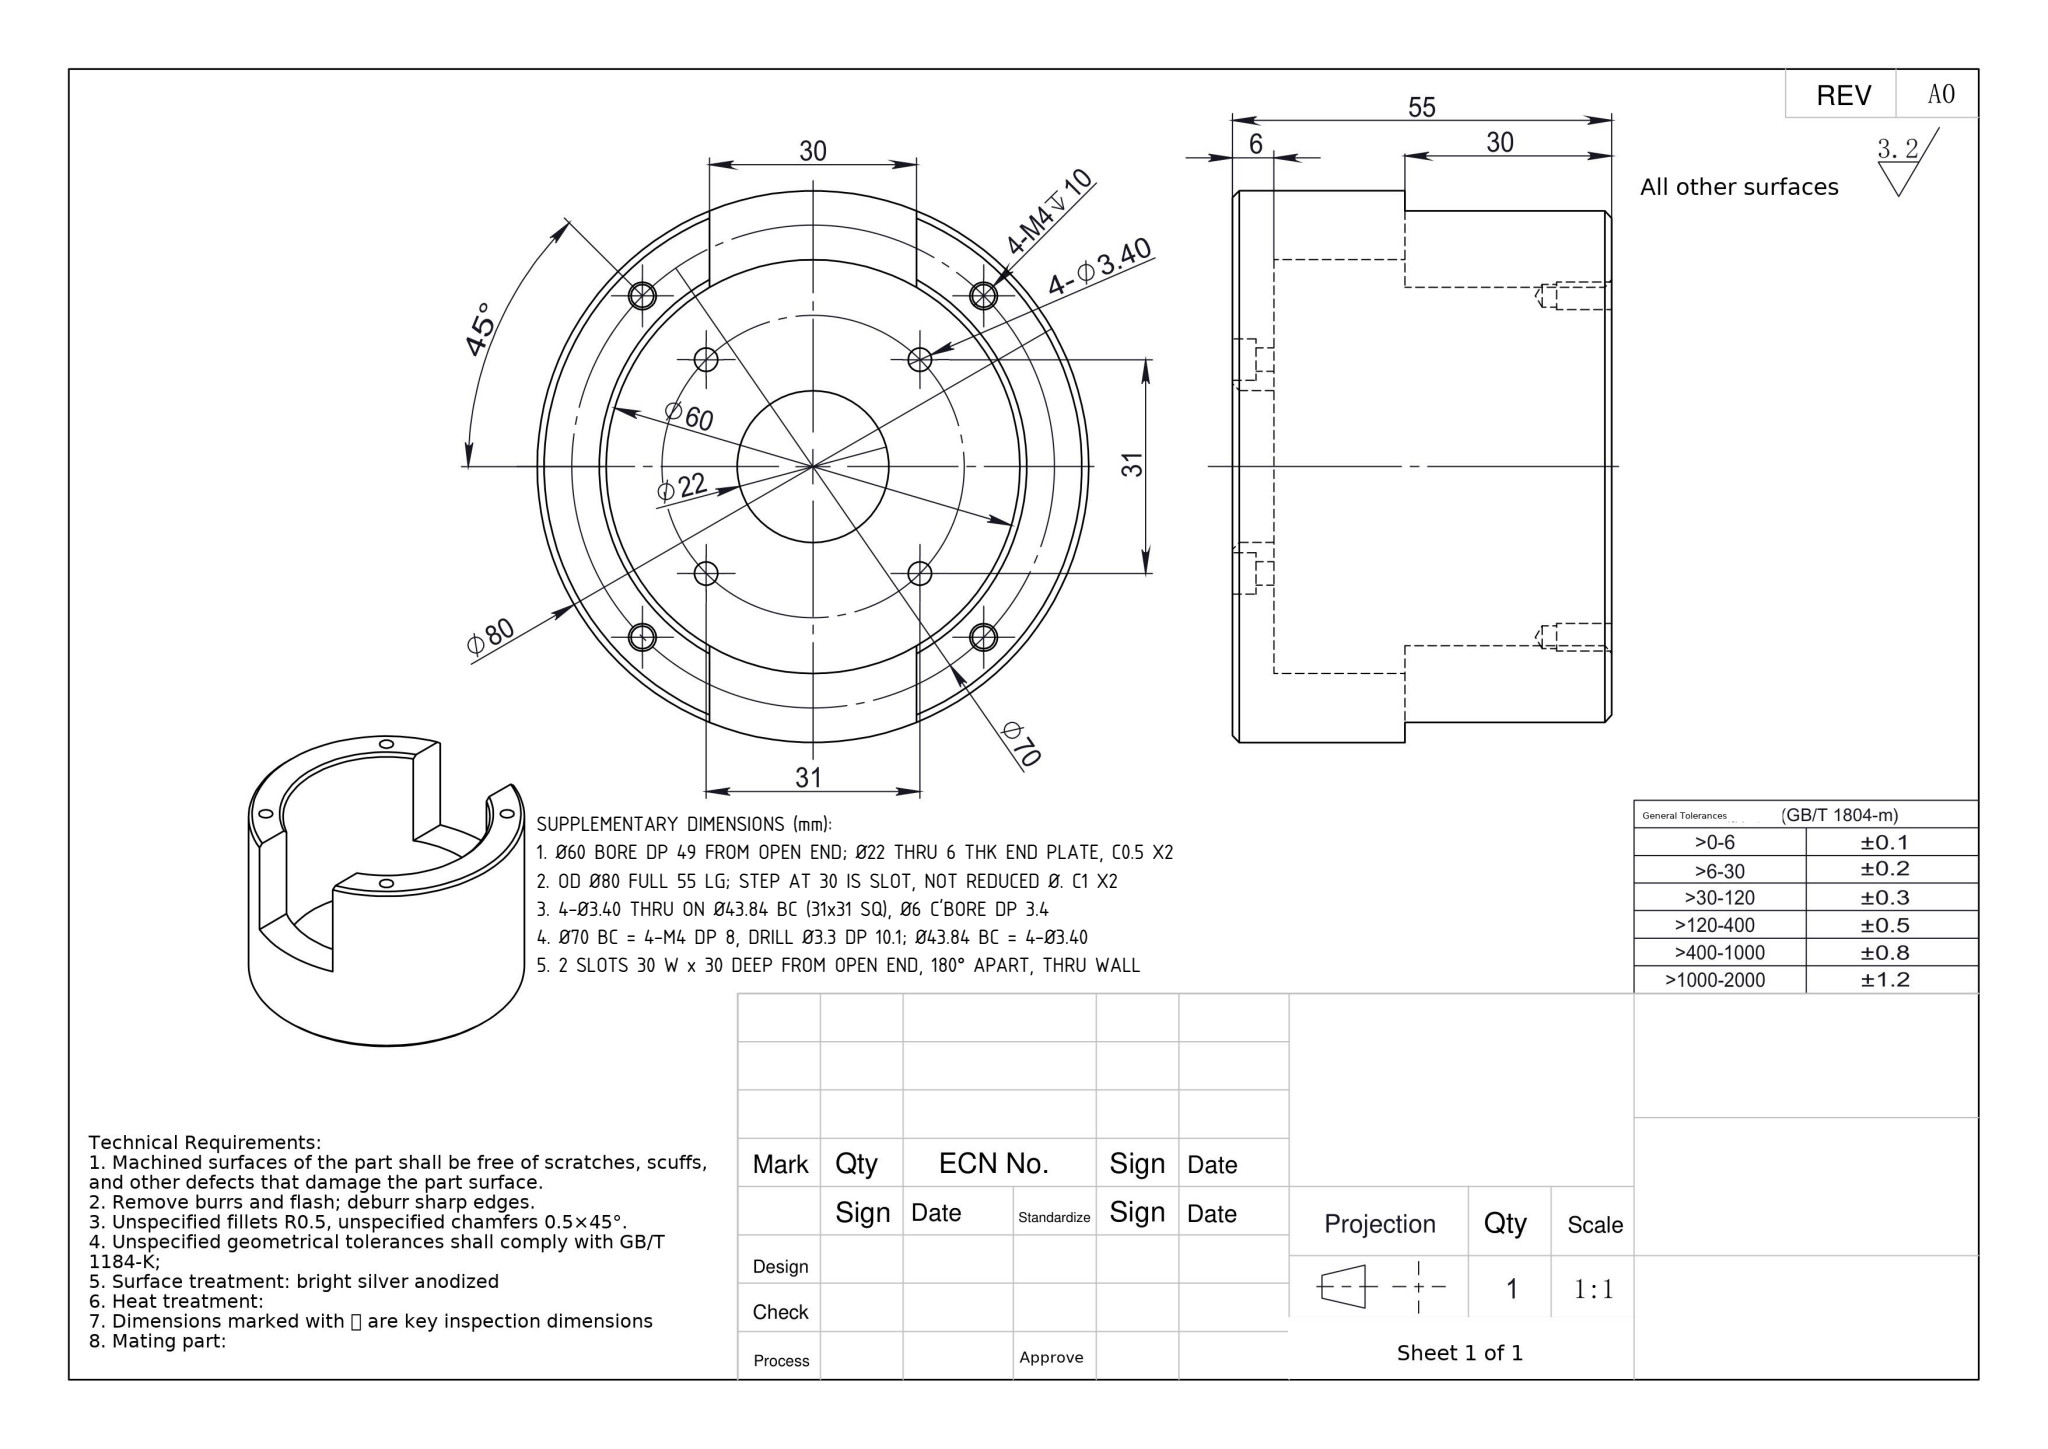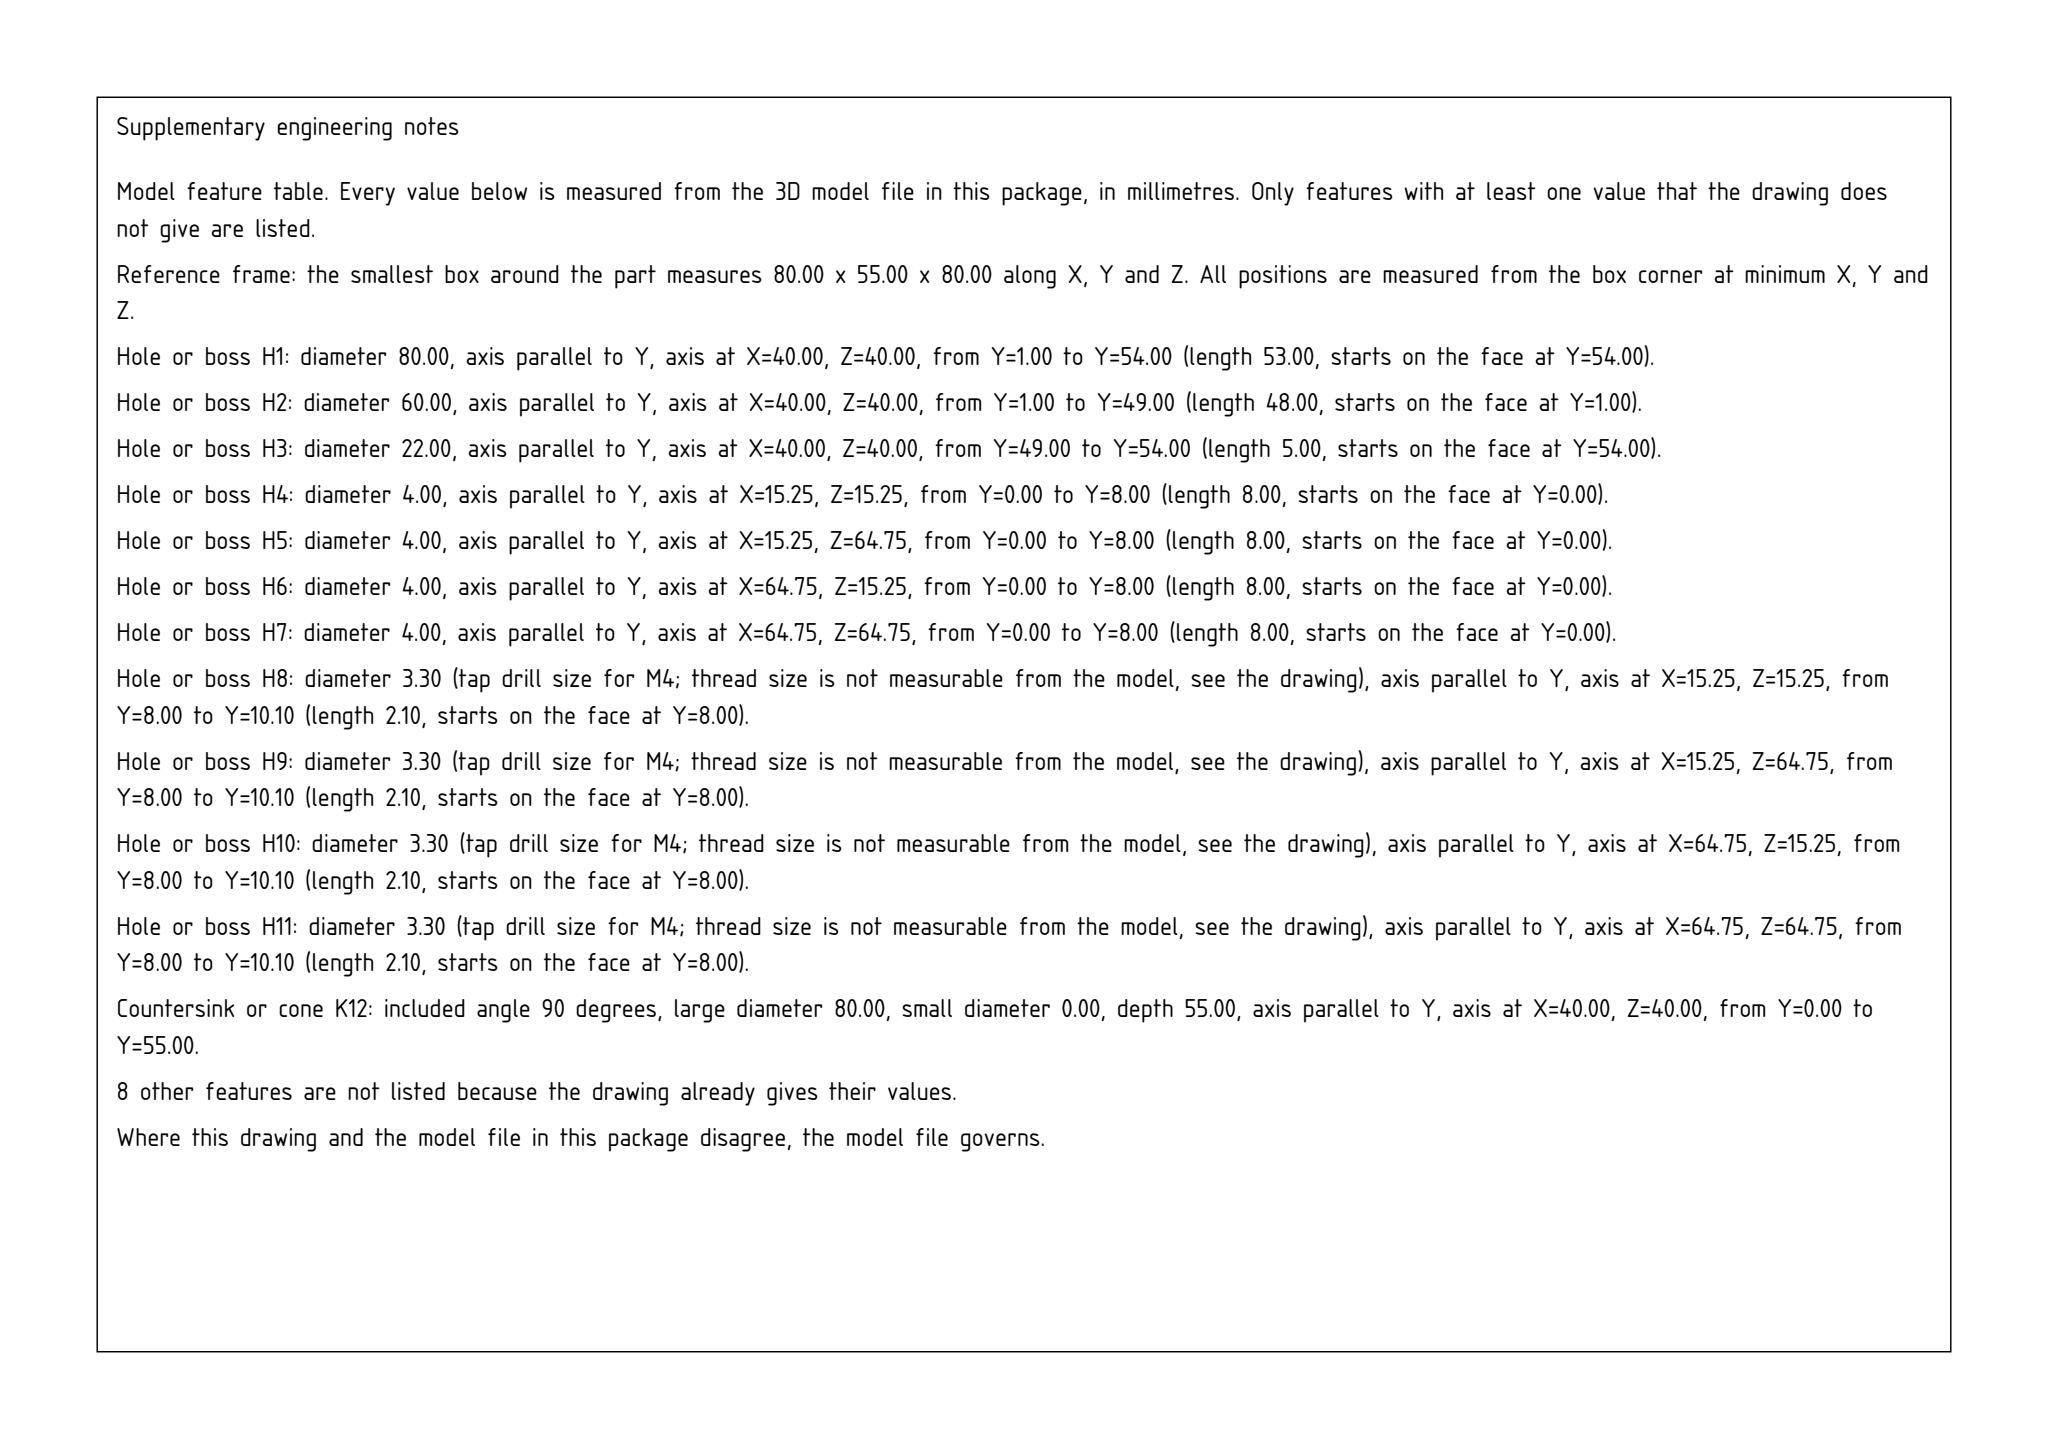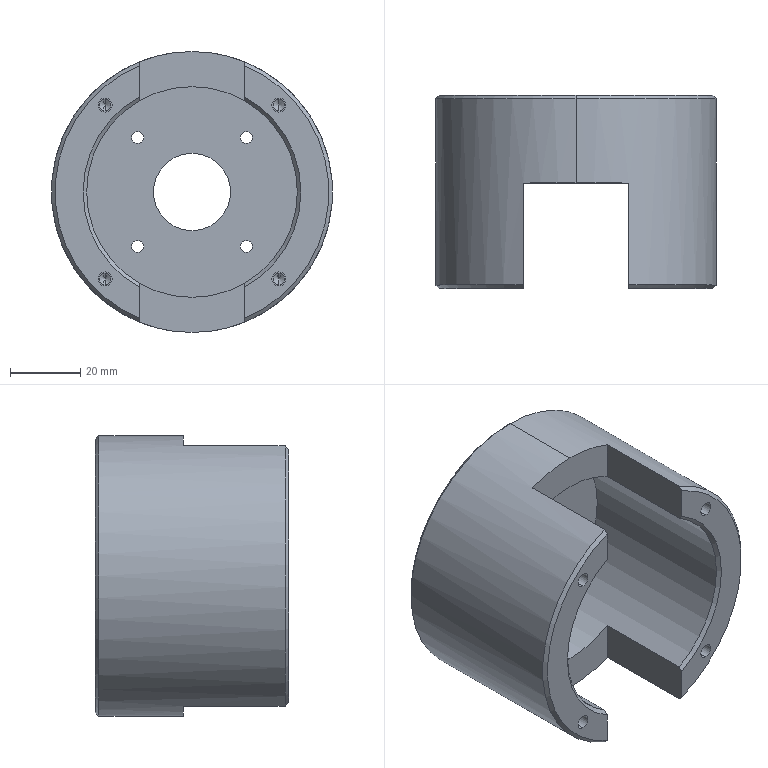Part | SolidWorks | mm | 1 solid | 72 faces | box 80 x 55 x 80 mm | volume 115735 mm3 | cylinder 38 | plane 18 | cone 16 | commonest cylinder face diameters 4 x8 3.3 x8 6 x8 3.4 x8 22 x2 60 x2 80 x2
build123d program:
from build123d import *

# Parameters (mm, degrees)
SKETCH1_R                                         = 40
EXTRUDE1_DEPTH                                    = 55
SKETCH1_2_R                                       = 30
CUT_EXTRUDE1_DEPTH                                = 49
HOLE_SIZE_ACCORDING_TO_TYPE_OF_HEXAGO_D           = 3.4
HOLE_SIZE_ACCORDING_TO_TYPE_OF_HEXAGO_DEPTH       = 35
HOLE_SIZE_ACCORDING_TO_TYPE_OF_HEXAGO_CBORE_D     = 6
HOLE_SIZE_ACCORDING_TO_TYPE_OF_HEXAGO_CBORE_DEPTH = 3.4
HOLE_SIZE_ACCORDING_TO_TYPE_OF_HEXAGO_TIP         = 1.021
SKETCH2_R                                         = 11
CUT_EXTRUDE2_DEPTH                                = 79.899
CHAMFER1_SIZE                                     = 1
SKETCH3_2_W                                       = 30
SKETCH3_2_H                                       = 89.726
CUT_EXTRUDE3_DEPTH                                = 30
M4_TAPPED_HOLE1_D                                 = 3.3
M4_TAPPED_HOLE1_DEPTH                             = 10.1
M4_TAPPED_HOLE1_CBORE_D                           = 4
M4_TAPPED_HOLE1_CBORE_DEPTH                       = 8
M4_TAPPED_HOLE1_TIP                               = 0.9914


with BuildPart() as part:
    # Sketch1 → Extrude1 (new body)
    with BuildSketch(Plane(origin=(0, 0, 0), x_dir=(1, 0, 0), z_dir=(0, 1, 0))):
        with Locations(Location((0, 0, 0), (0, 0, 270))):
            Circle(SKETCH1_R)
    extrude(amount=EXTRUDE1_DEPTH)

    # Sketch1_2 → Cut-Extrude1 (cut)
    with BuildSketch(Plane.XZ):
        with Locations(Location((0, 0, 0), (0, 0, 270))):
            Circle(SKETCH1_2_R)
    extrude(amount=-CUT_EXTRUDE1_DEPTH, mode=Mode.SUBTRACT)

    # Hole Size _ according to_ Type of Hexago
    with Locations(Plane(origin=(0, 55, 0), x_dir=(1, 0, 0), z_dir=(0, 1, 0))):
        with Locations((-15.5, 15.5), (15.5, 15.5), (15.5, -15.5), (-15.5, -15.5)):
            CounterBoreHole(HOLE_SIZE_ACCORDING_TO_TYPE_OF_HEXAGO_D / 2, HOLE_SIZE_ACCORDING_TO_TYPE_OF_HEXAGO_CBORE_D / 2, HOLE_SIZE_ACCORDING_TO_TYPE_OF_HEXAGO_CBORE_DEPTH, depth=HOLE_SIZE_ACCORDING_TO_TYPE_OF_HEXAGO_DEPTH)
            with Locations((0, 0, -(HOLE_SIZE_ACCORDING_TO_TYPE_OF_HEXAGO_DEPTH + HOLE_SIZE_ACCORDING_TO_TYPE_OF_HEXAGO_TIP / 2))):  # 118° drill point
                Cone(0, HOLE_SIZE_ACCORDING_TO_TYPE_OF_HEXAGO_D / 2, HOLE_SIZE_ACCORDING_TO_TYPE_OF_HEXAGO_TIP, mode=Mode.SUBTRACT)

    # Sketch2 → Cut-Extrude2 (cut, through all)
    with BuildSketch(Plane(origin=(0, 55, 0), x_dir=(1, 0, 0), z_dir=(0, 1, 0))):
        with Locations(Location((0, 0, 0), (0, 0, 270))):
            Circle(SKETCH2_R)
    extrude(amount=-CUT_EXTRUDE2_DEPTH, mode=Mode.SUBTRACT)

    # Chamfer1
    chamfer1_edges = [part.edges().sort_by_distance(p)[0] for p in [
        (0, 0, -40),
        (0, 55, -40),
        (0, 55, -11),
        (0, 0, 30),
    ]]
    chamfer(chamfer1_edges, length=CHAMFER1_SIZE)

    # Sketch3_2 → Cut-Extrude3 (cut)
    with BuildSketch(Plane.XZ):
        Rectangle(SKETCH3_2_W, SKETCH3_2_H)
    extrude(amount=-CUT_EXTRUDE3_DEPTH, mode=Mode.SUBTRACT)

    # M4 Tapped Hole1
    with Locations(Plane.XZ):
        with Locations((-24.749, 24.749), (-24.749, -24.749), (24.749, -24.749), (24.749, 24.749)):
            CounterBoreHole(M4_TAPPED_HOLE1_D / 2, M4_TAPPED_HOLE1_CBORE_D / 2, M4_TAPPED_HOLE1_CBORE_DEPTH, depth=M4_TAPPED_HOLE1_DEPTH)
            with Locations((0, 0, -(M4_TAPPED_HOLE1_DEPTH + M4_TAPPED_HOLE1_TIP / 2))):  # 118° drill point
                Cone(0, M4_TAPPED_HOLE1_D / 2, M4_TAPPED_HOLE1_TIP, mode=Mode.SUBTRACT)


solid = part.part